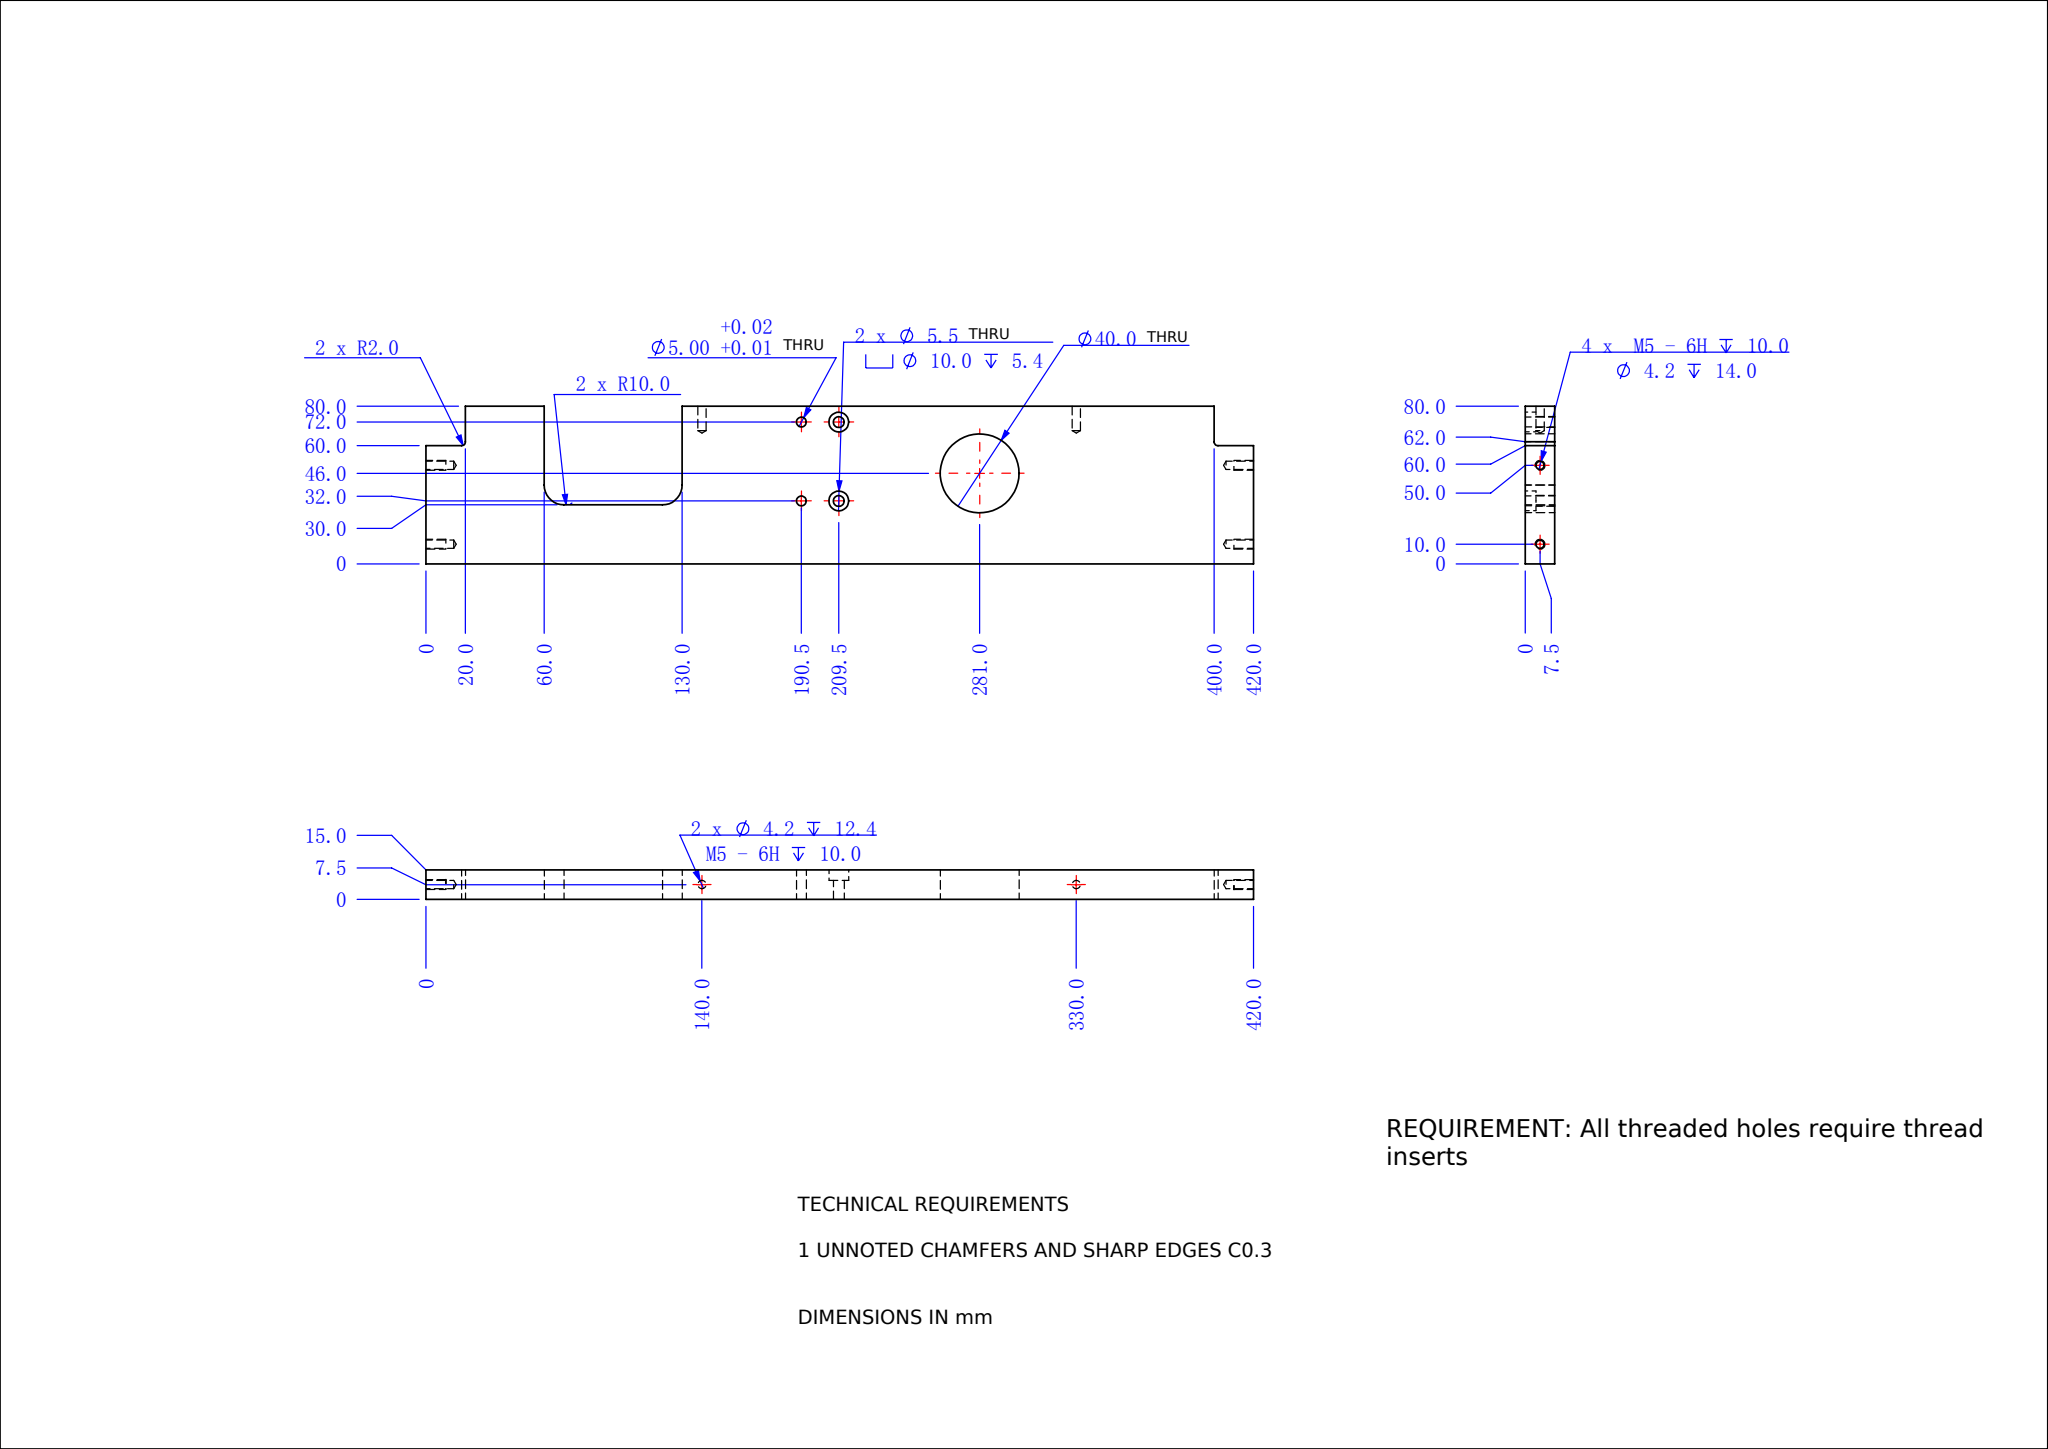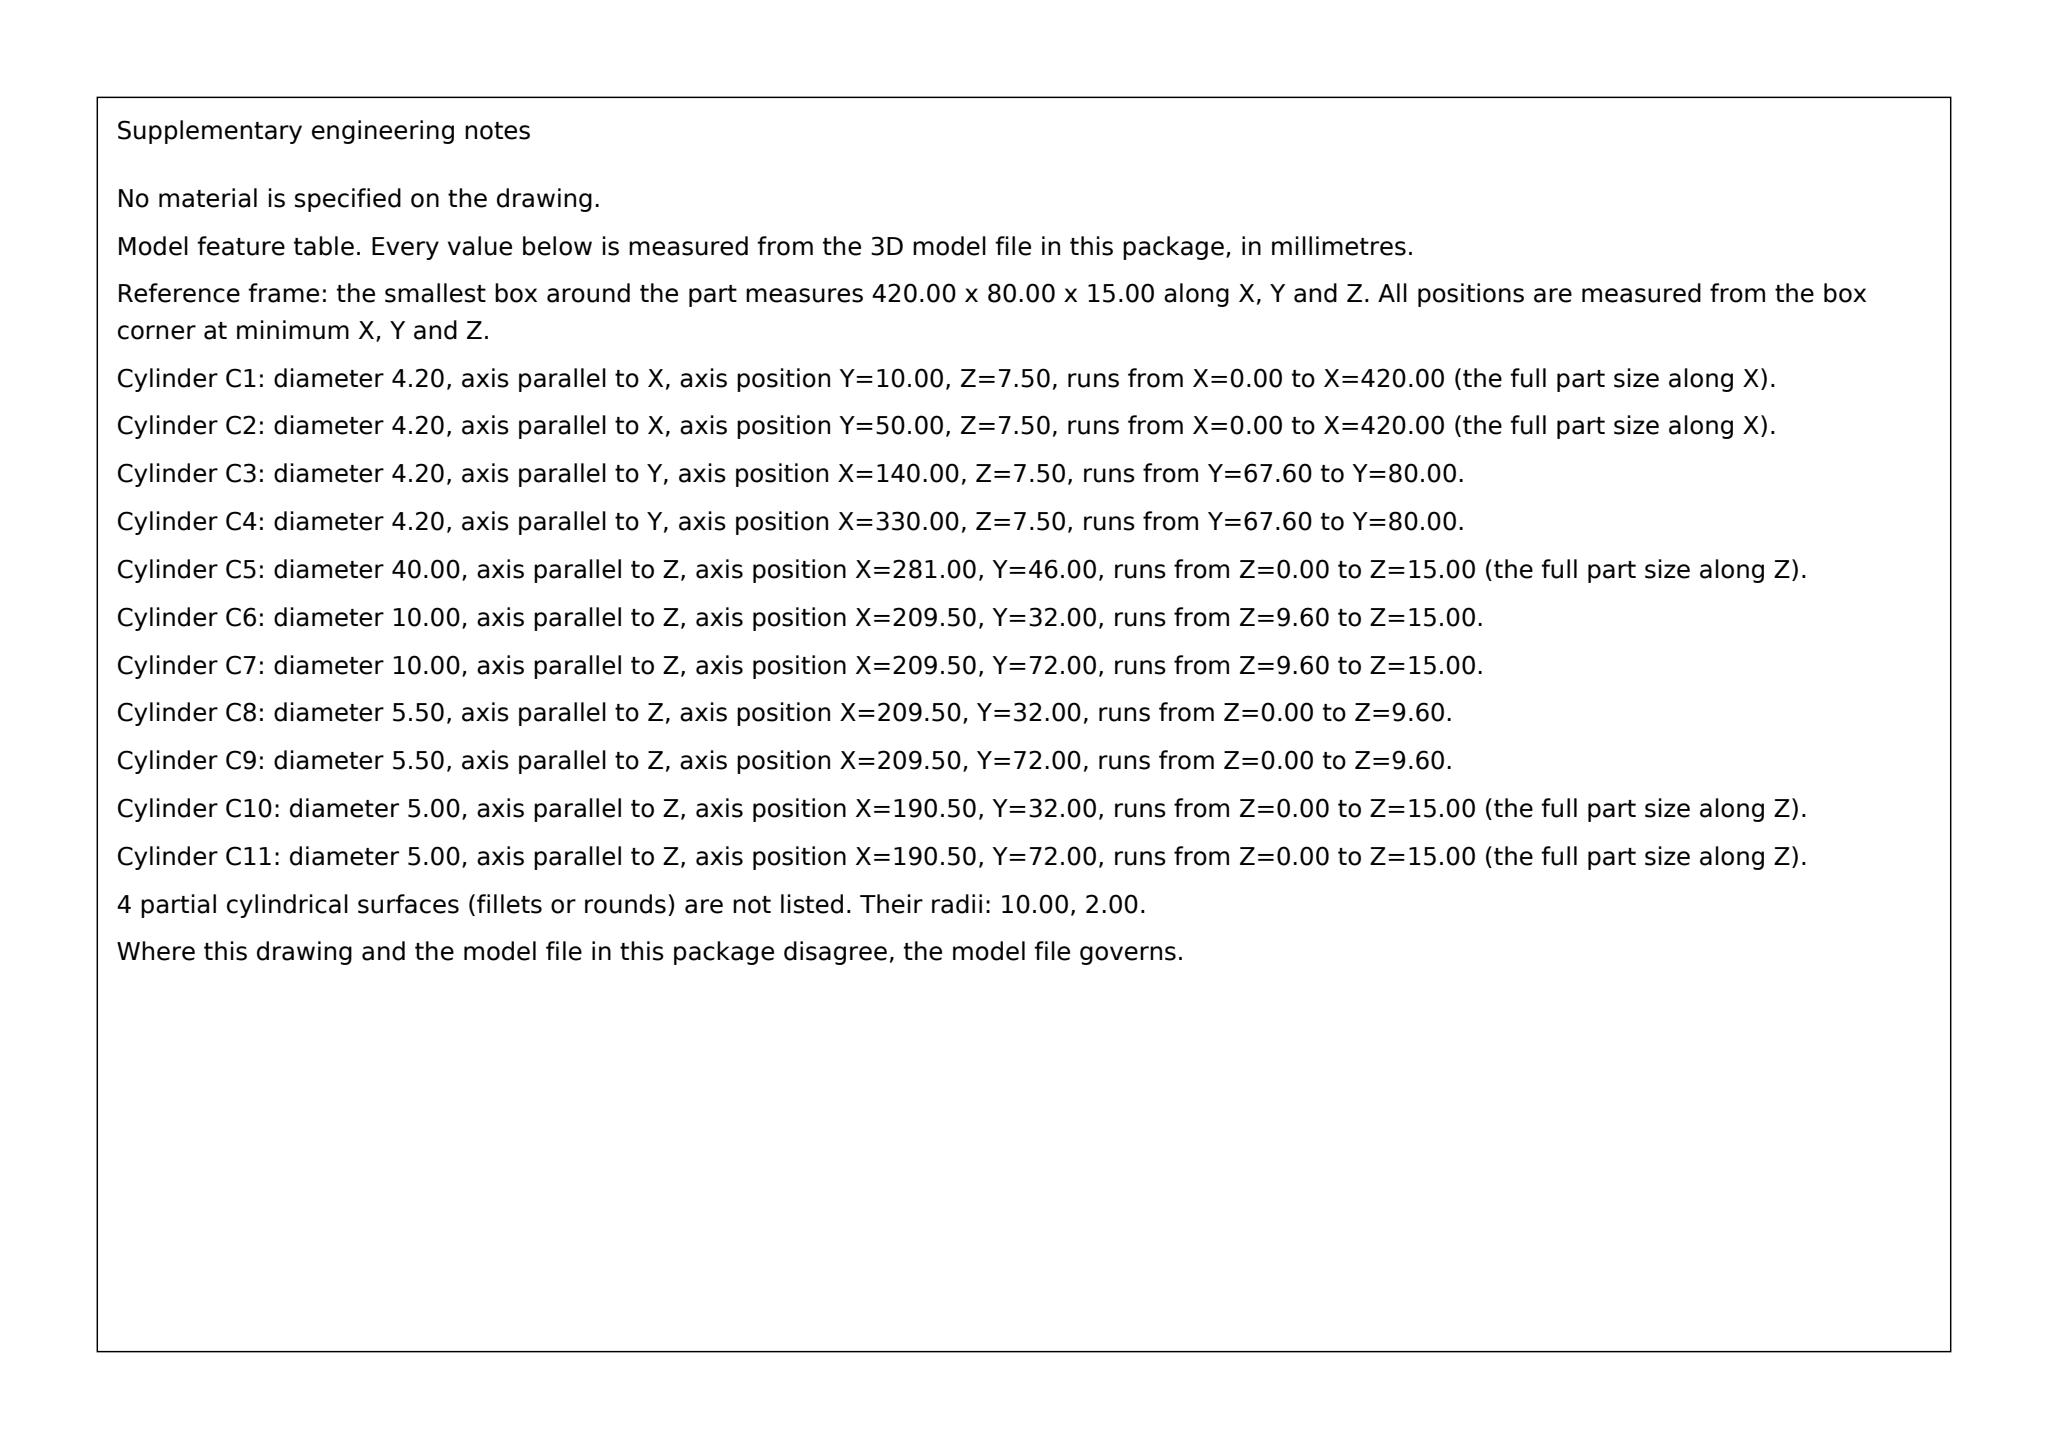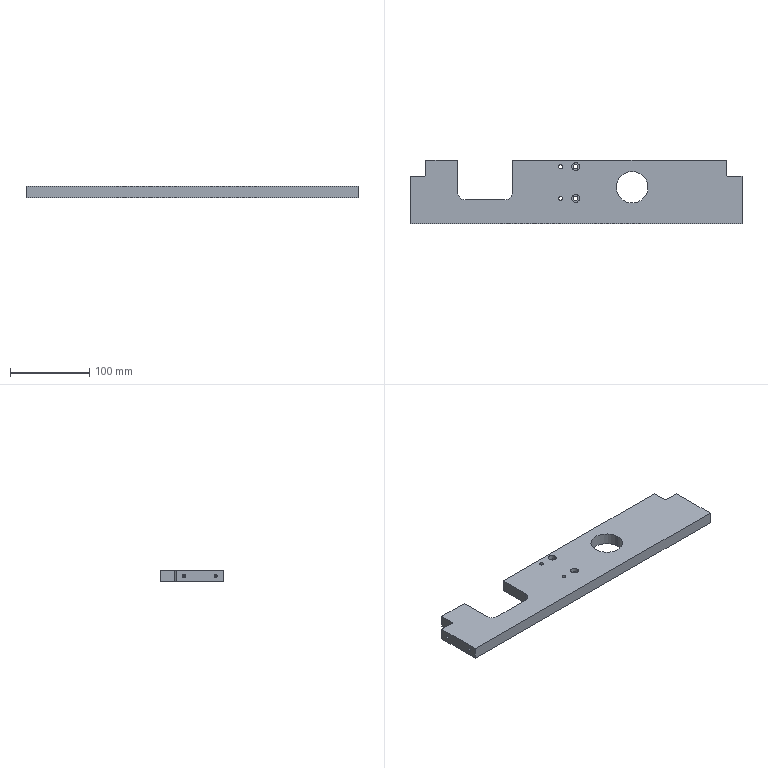Part | SolidWorks | mm | 1 solid | 58 faces | box 420 x 80 x 15 mm | volume 418272 mm3 | cylinder 30 | plane 16 | cone 12 | commonest cylinder face diameters 4.2 x12 5 x4 10 x4 5.5 x4 40 x2 4 x2 20 x2
build123d program:
from build123d import *

# Parameters (mm, degrees)
SKETCH1_R                                       = 20
BOSS_EXTRUDE1_DEPTH                             = 15
FILLET1_R                                       = 2
M5_TAPPED_HOLE1_D                               = 4.2
M5_TAPPED_HOLE1_DEPTH                           = 14
M5_TAPPED_HOLE1_TIP                             = 1.262
M5_TAPPED_HOLE2_D                               = 4.2
M5_TAPPED_HOLE2_DEPTH                           = 14
M5_TAPPED_HOLE2_TIP                             = 1.262
M5_HEX_SOCKET_HEAD_CAP_SCREW_CBORE1_D           = 5.5
M5_HEX_SOCKET_HEAD_CAP_SCREW_CBORE1_CBORE_D     = 10
M5_HEX_SOCKET_HEAD_CAP_SCREW_CBORE1_CBORE_DEPTH = 5.4
LPATTERN1_COUNT                                 = 2
LPATTERN1_PITCH                                 = 40
SKETCH12_R                                      = 2.5
CUT_EXTRUDE1_DEPTH                              = 428.814
SKETCH15_W                                      = 70
SKETCH15_H                                      = 50
CUT_EXTRUDE2_DEPTH                              = 428.814
FILLET2_R                                       = 10
M5_TAPPED_HOLE3_D                               = 4.2
M5_TAPPED_HOLE3_DEPTH                           = 12.4
M5_TAPPED_HOLE3_TIP                             = 1.262


with BuildPart() as part:
    # Sketch1 → Boss-Extrude1 (new body)
    with BuildSketch(Plane.XY):
        Polygon((0, 0), (420, 0), (420, 60), (400, 60), (400, 80), (20, 80), (20, 60), (0, 60), align=None)
        with Locations((281, 46)):
            Circle(SKETCH1_R, mode=Mode.SUBTRACT)
    extrude(amount=BOSS_EXTRUDE1_DEPTH)

    # Fillet1
    fillet1_edges = [part.edges().sort_by_distance(p)[0] for p in [
        (20, 60, 7.5),
        (400, 60, 7.5),
    ]]
    fillet(fillet1_edges, radius=FILLET1_R)

    # M5 Tapped Hole1
    with Locations(Plane.ZY):
        with Locations((7.5, 50), (7.5, 10)):
            Hole(M5_TAPPED_HOLE1_D / 2, depth=M5_TAPPED_HOLE1_DEPTH)
            with Locations((0, 0, -(M5_TAPPED_HOLE1_DEPTH + M5_TAPPED_HOLE1_TIP / 2))):  # 118° drill point
                Cone(0, M5_TAPPED_HOLE1_D / 2, M5_TAPPED_HOLE1_TIP, mode=Mode.SUBTRACT)

    # M5 Tapped Hole2
    with Locations(Plane(origin=(420, 0, 0), x_dir=(0, 0, -1), z_dir=(1, 0, 0))):
        with Locations((-7.5, 50), (-7.5, 10)):
            Hole(M5_TAPPED_HOLE2_D / 2, depth=M5_TAPPED_HOLE2_DEPTH)
            with Locations((0, 0, -(M5_TAPPED_HOLE2_DEPTH + M5_TAPPED_HOLE2_TIP / 2))):  # 118° drill point
                Cone(0, M5_TAPPED_HOLE2_D / 2, M5_TAPPED_HOLE2_TIP, mode=Mode.SUBTRACT)

    # M5 Hex Socket Head Cap Screw CBORE1 (through all)
    with Locations(Plane.XY.offset(15)):
        with Locations((209.5, 32)):
            m5_hex_socket_head_cap_screw_cbore1 = CounterBoreHole(M5_HEX_SOCKET_HEAD_CAP_SCREW_CBORE1_D / 2, M5_HEX_SOCKET_HEAD_CAP_SCREW_CBORE1_CBORE_D / 2, M5_HEX_SOCKET_HEAD_CAP_SCREW_CBORE1_CBORE_DEPTH)

    # LPattern1: M5 Hex Socket Head Cap Screw CBORE1 ×2
    with Locations(*[(0, i * LPATTERN1_PITCH, 0) for i in range(1, LPATTERN1_COUNT)]):
        add(m5_hex_socket_head_cap_screw_cbore1, mode=Mode.SUBTRACT)

    # Sketch12 → Cut-Extrude1 (cut, through all)
    with BuildSketch(Plane.XY.offset(15)):
        with Locations((190.5, 72)):
            Circle(SKETCH12_R)
        with Locations((190.5, 32)):
            Circle(SKETCH12_R)
    extrude(amount=-CUT_EXTRUDE1_DEPTH, mode=Mode.SUBTRACT)

    # Sketch15 → Cut-Extrude2 (cut, through all)
    with BuildSketch(Plane.XY.offset(15)):
        with Locations((95, 55)):
            Rectangle(SKETCH15_W, SKETCH15_H)
    extrude(amount=-CUT_EXTRUDE2_DEPTH, mode=Mode.SUBTRACT)

    # Fillet2
    fillet2_edges = [part.edges().sort_by_distance(p)[0] for p in [
        (60, 30, 7.5),
        (130, 30, 7.5),
    ]]
    fillet(fillet2_edges, radius=FILLET2_R)

    # M5 Tapped Hole3
    with Locations(Plane(origin=(0, 80, 0), x_dir=(1, 0, 0), z_dir=(0, 1, 0))):
        with Locations((330, -7.5), (140, -7.5)):
            Hole(M5_TAPPED_HOLE3_D / 2, depth=M5_TAPPED_HOLE3_DEPTH)
            with Locations((0, 0, -(M5_TAPPED_HOLE3_DEPTH + M5_TAPPED_HOLE3_TIP / 2))):  # 118° drill point
                Cone(0, M5_TAPPED_HOLE3_D / 2, M5_TAPPED_HOLE3_TIP, mode=Mode.SUBTRACT)


solid = part.part